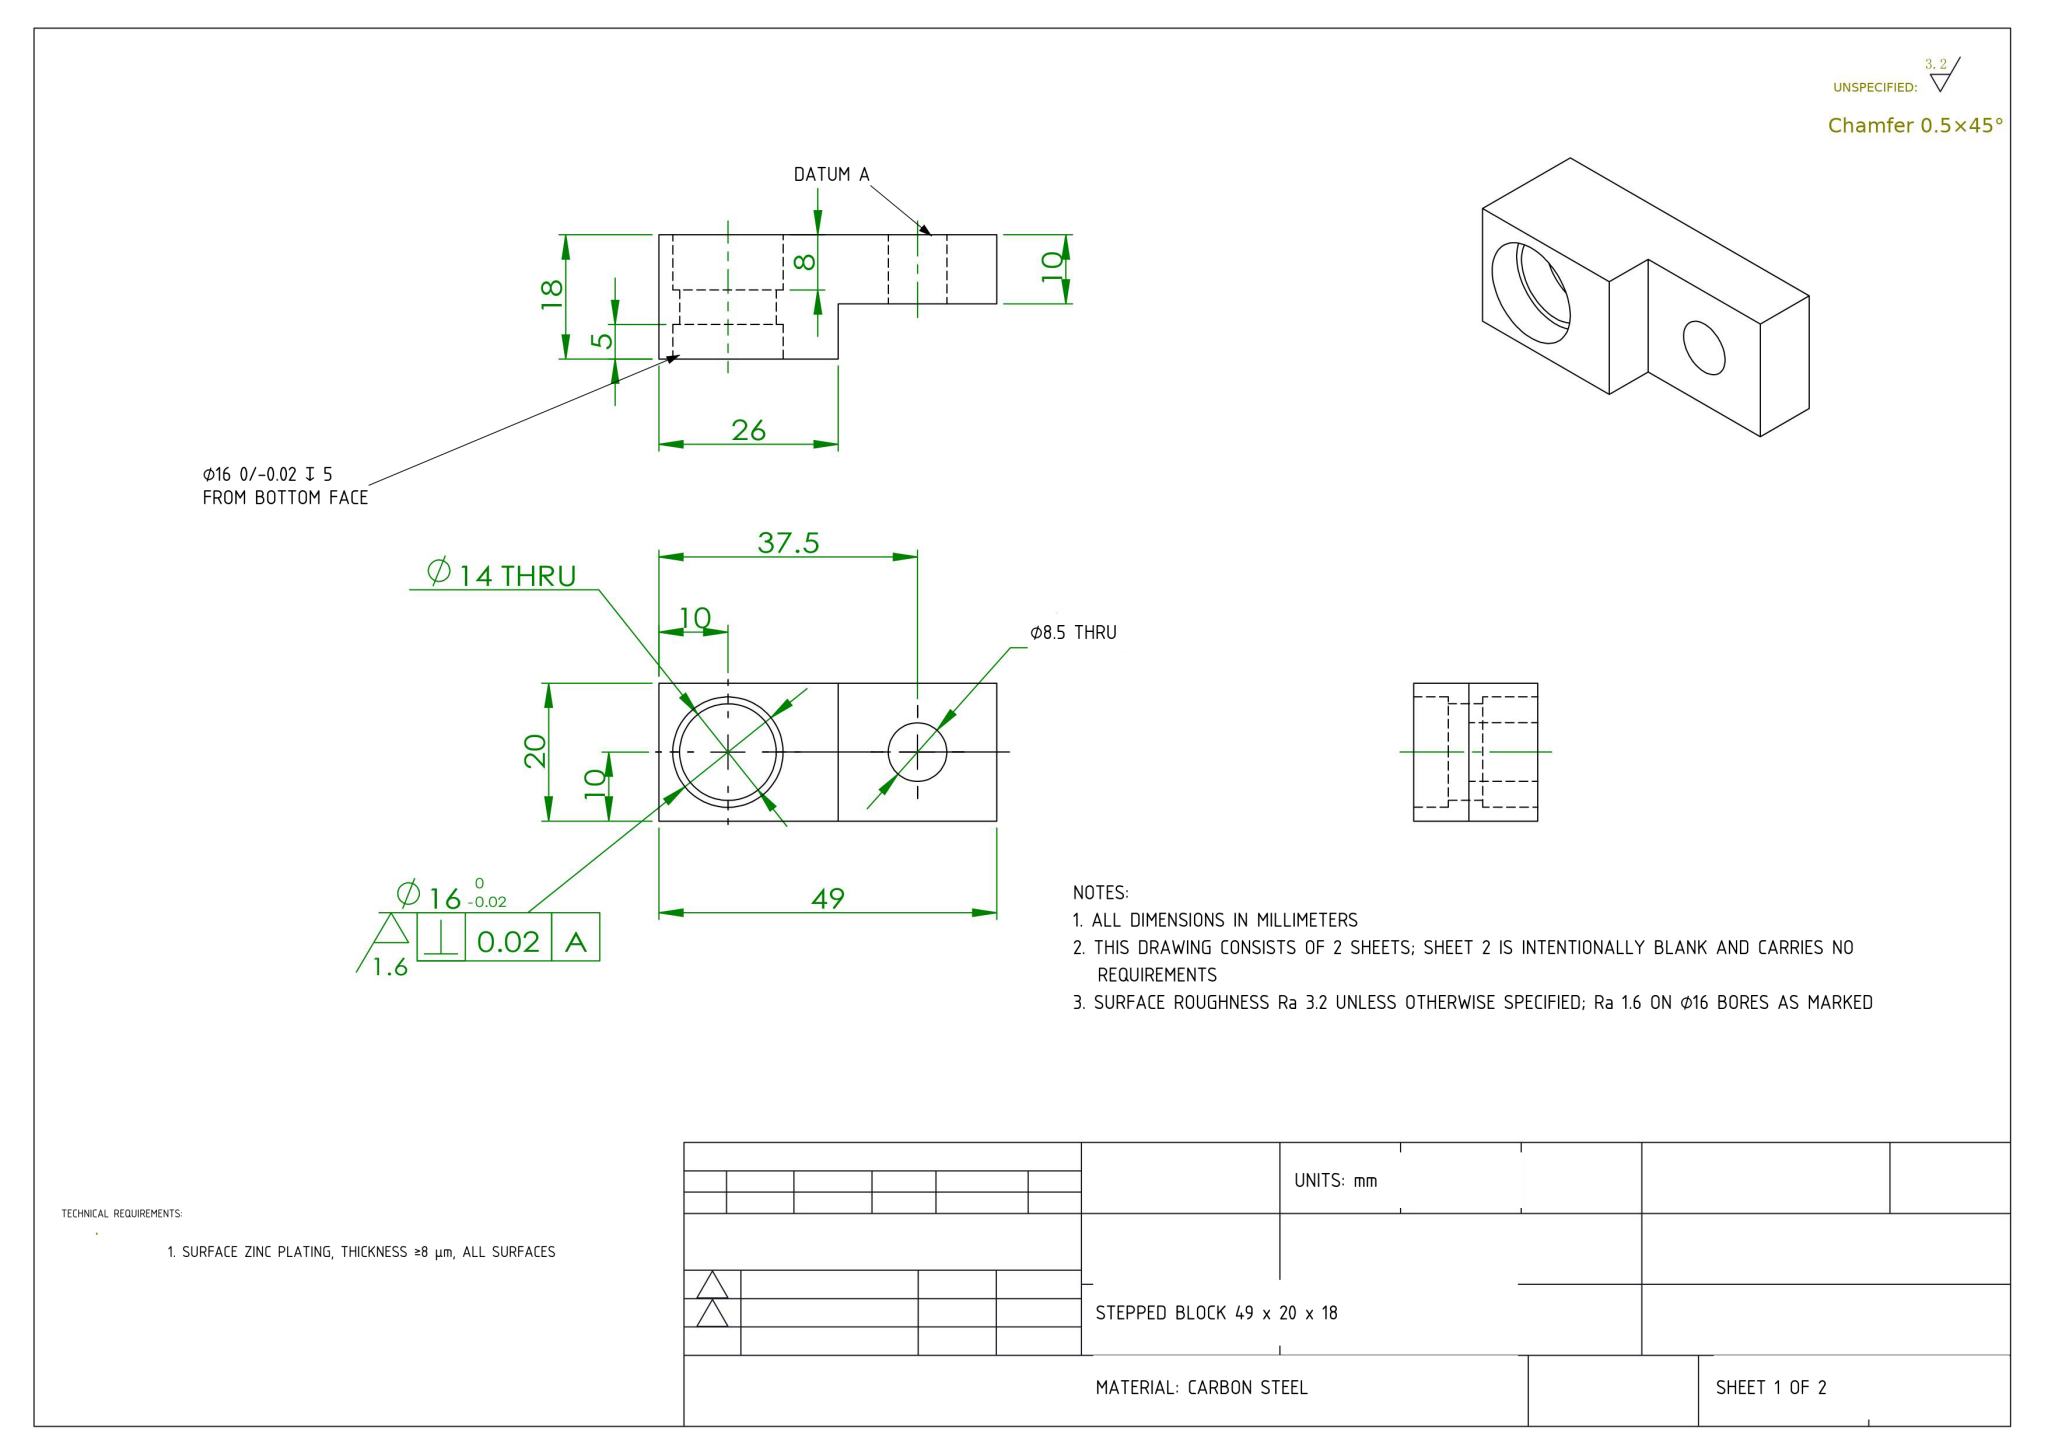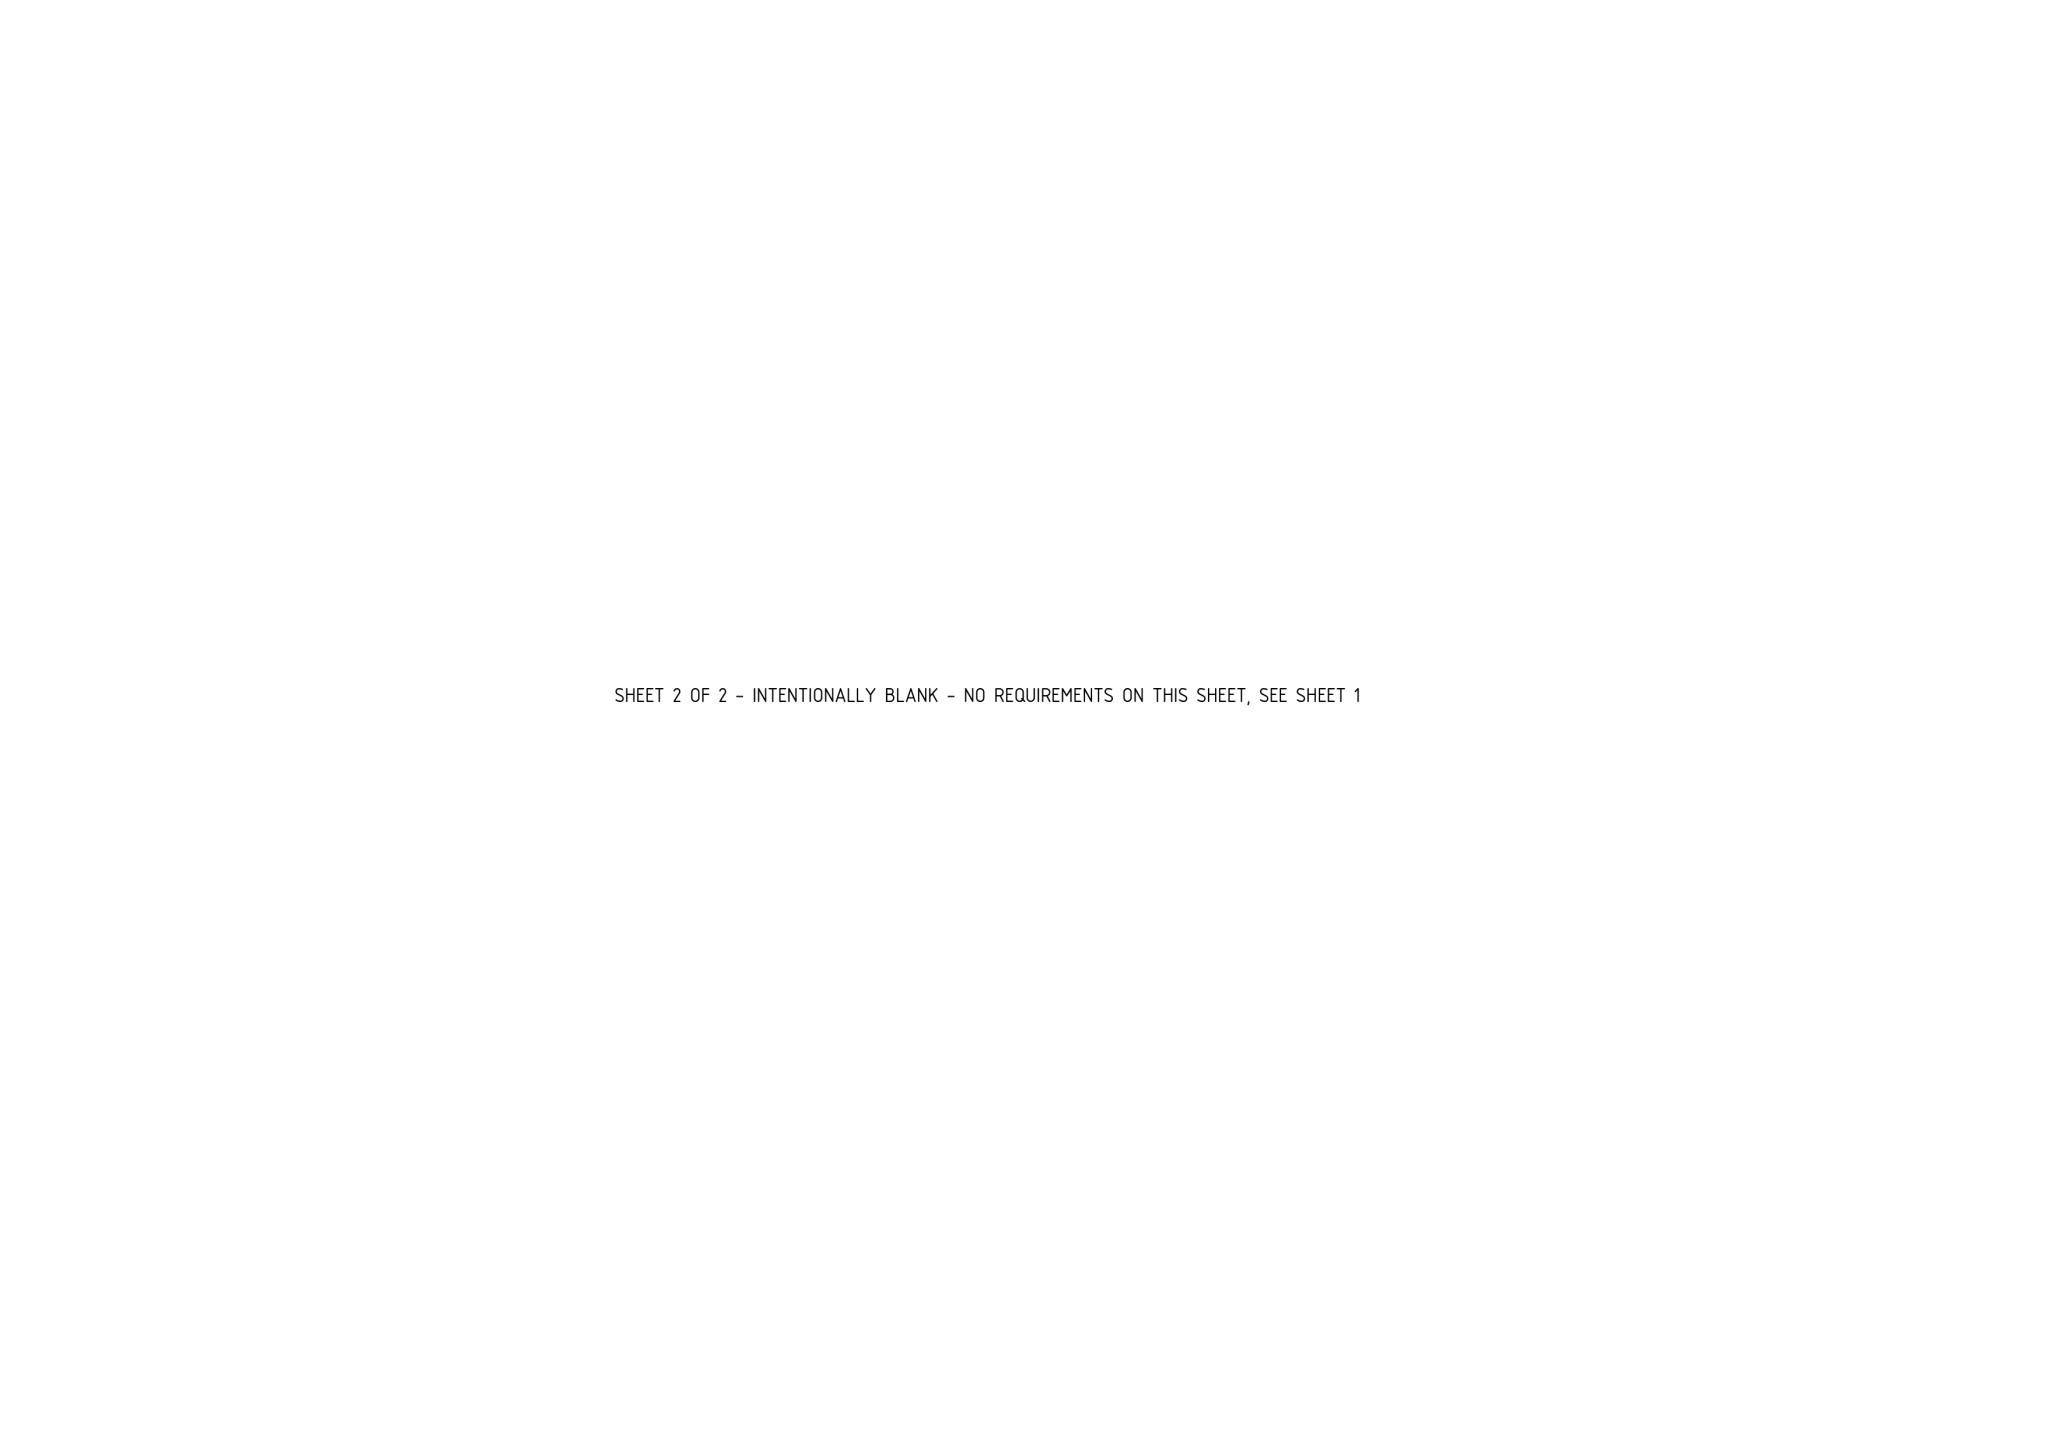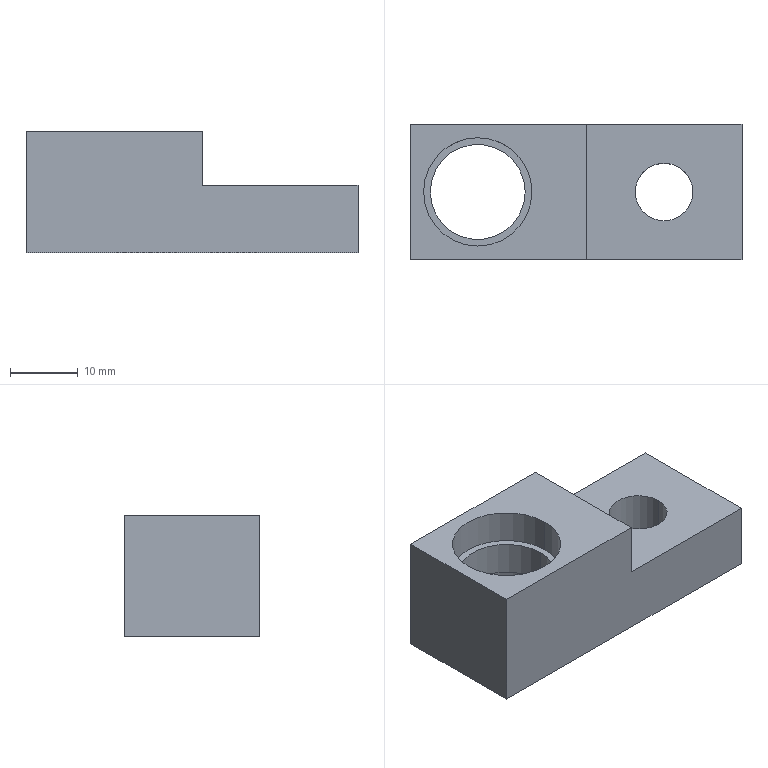Part | NX | mm | 1 solid | 18 faces | box 49 x 20 x 18 mm | volume 10009 mm3 | plane 10 | cylinder 8 | commonest cylinder face diameters 16 x4 8.5 x2 14 x2
STEP:
#1=COLOUR_RGB('',0.7961,0.8235,0.9373);
#2=FILL_AREA_STYLE_COLOUR('',#1);
#3=FILL_AREA_STYLE('',(#2));
#4=SURFACE_STYLE_FILL_AREA(#3);
#5=SURFACE_SIDE_STYLE('',(#4));
#6=SURFACE_STYLE_USAGE(.BOTH.,#5);
#7=PRESENTATION_STYLE_ASSIGNMENT((#6));
#8=CARTESIAN_POINT('',(18.,0.,8.));
#9=VERTEX_POINT('',#8);
#10=CARTESIAN_POINT('',(2.,0.,8.));
#11=VERTEX_POINT('',#10);
#12=CARTESIAN_POINT('',(10.,0.,8.));
#13=DIRECTION('',(0.,0.,-1.));
#14=DIRECTION('',(-1.,0.,0.));
#15=AXIS2_PLACEMENT_3D('',#12,#13,#14);
#16=CIRCLE('',#15,8.);
#17=EDGE_CURVE('',#9,#11,#16,.T.);
#18=ORIENTED_EDGE('',*,*,#17,.F.);
#19=CARTESIAN_POINT('',(18.,0.,0.));
#20=VERTEX_POINT('',#19);
#21=CARTESIAN_POINT('',(18.,0.,8.));
#22=DIRECTION('',(0.,0.,-1.));
#23=VECTOR('',#22,1000.);
#24=LINE('',#21,#23);
#25=EDGE_CURVE('',#9,#20,#24,.T.);
#26=ORIENTED_EDGE('',*,*,#25,.T.);
#27=CARTESIAN_POINT('',(2.,0.,0.));
#28=VERTEX_POINT('',#27);
#29=CARTESIAN_POINT('',(10.,0.,0.));
#30=DIRECTION('',(0.,0.,-1.));
#31=DIRECTION('',(-1.,0.,0.));
#32=AXIS2_PLACEMENT_3D('',#29,#30,#31);
#33=CIRCLE('',#32,8.);
#34=EDGE_CURVE('',#20,#28,#33,.T.);
#35=ORIENTED_EDGE('',*,*,#34,.T.);
#36=CARTESIAN_POINT('',(2.,0.,8.));
#37=DIRECTION('',(0.,0.,-1.));
#38=VECTOR('',#37,1000.);
#39=LINE('',#36,#38);
#40=EDGE_CURVE('',#11,#28,#39,.T.);
#41=ORIENTED_EDGE('',*,*,#40,.F.);
#42=EDGE_LOOP('',(#18,#26,#35,#41));
#43=FACE_OUTER_BOUND('',#42,.T.);
#44=CARTESIAN_POINT('',(10.,0.,8.));
#45=DIRECTION('',(0.,0.,-1.));
#46=DIRECTION('',(-1.,0.,0.));
#47=AXIS2_PLACEMENT_3D('',#44,#45,#46);
#48=CYLINDRICAL_SURFACE('',#47,8.);
#49=ADVANCED_FACE('',(#43),#48,.F.);
#50=CARTESIAN_POINT('',(2.,0.,13.));
#51=VERTEX_POINT('',#50);
#52=CARTESIAN_POINT('',(18.,0.,13.));
#53=VERTEX_POINT('',#52);
#54=CARTESIAN_POINT('',(10.,0.,13.));
#55=DIRECTION('',(0.,0.,1.));
#56=DIRECTION('',(1.,0.,0.));
#57=AXIS2_PLACEMENT_3D('',#54,#55,#56);
#58=CIRCLE('',#57,8.);
#59=EDGE_CURVE('',#51,#53,#58,.T.);
#60=ORIENTED_EDGE('',*,*,#59,.F.);
#61=CARTESIAN_POINT('',(2.,0.,18.));
#62=VERTEX_POINT('',#61);
#63=CARTESIAN_POINT('',(2.,0.,13.));
#64=DIRECTION('',(0.,0.,1.));
#65=VECTOR('',#64,1000.);
#66=LINE('',#63,#65);
#67=EDGE_CURVE('',#51,#62,#66,.T.);
#68=ORIENTED_EDGE('',*,*,#67,.T.);
#69=CARTESIAN_POINT('',(18.,0.,18.));
#70=VERTEX_POINT('',#69);
#71=CARTESIAN_POINT('',(10.,0.,18.));
#72=DIRECTION('',(0.,0.,1.));
#73=DIRECTION('',(1.,0.,0.));
#74=AXIS2_PLACEMENT_3D('',#71,#72,#73);
#75=CIRCLE('',#74,8.);
#76=EDGE_CURVE('',#62,#70,#75,.T.);
#77=ORIENTED_EDGE('',*,*,#76,.T.);
#78=CARTESIAN_POINT('',(18.,0.,13.));
#79=DIRECTION('',(0.,0.,1.));
#80=VECTOR('',#79,1000.);
#81=LINE('',#78,#80);
#82=EDGE_CURVE('',#53,#70,#81,.T.);
#83=ORIENTED_EDGE('',*,*,#82,.F.);
#84=EDGE_LOOP('',(#60,#68,#77,#83));
#85=FACE_OUTER_BOUND('',#84,.T.);
#86=CARTESIAN_POINT('',(10.,0.,13.));
#87=DIRECTION('',(0.,0.,1.));
#88=DIRECTION('',(1.,0.,0.));
#89=AXIS2_PLACEMENT_3D('',#86,#87,#88);
#90=CYLINDRICAL_SURFACE('',#89,8.);
#91=ADVANCED_FACE('',(#85),#90,.F.);
#92=CARTESIAN_POINT('',(33.25,0.,0.));
#93=VERTEX_POINT('',#92);
#94=CARTESIAN_POINT('',(41.75,0.,0.));
#95=VERTEX_POINT('',#94);
#96=CARTESIAN_POINT('',(37.5,0.,0.));
#97=DIRECTION('',(0.,0.,1.));
#98=DIRECTION('',(1.,0.,0.));
#99=AXIS2_PLACEMENT_3D('',#96,#97,#98);
#100=CIRCLE('',#99,4.25);
#101=EDGE_CURVE('',#93,#95,#100,.T.);
#102=ORIENTED_EDGE('',*,*,#101,.F.);
#103=CARTESIAN_POINT('',(33.25,0.,10.));
#104=VERTEX_POINT('',#103);
#105=CARTESIAN_POINT('',(33.25,0.,0.));
#106=DIRECTION('',(0.,0.,1.));
#107=VECTOR('',#106,1000.);
#108=LINE('',#105,#107);
#109=EDGE_CURVE('',#93,#104,#108,.T.);
#110=ORIENTED_EDGE('',*,*,#109,.T.);
#111=CARTESIAN_POINT('',(41.75,0.,10.));
#112=VERTEX_POINT('',#111);
#113=CARTESIAN_POINT('',(37.5,0.,10.));
#114=DIRECTION('',(0.,0.,1.));
#115=DIRECTION('',(1.,0.,0.));
#116=AXIS2_PLACEMENT_3D('',#113,#114,#115);
#117=CIRCLE('',#116,4.25);
#118=EDGE_CURVE('',#104,#112,#117,.T.);
#119=ORIENTED_EDGE('',*,*,#118,.T.);
#120=CARTESIAN_POINT('',(41.75,0.,0.));
#121=DIRECTION('',(0.,0.,1.));
#122=VECTOR('',#121,1000.);
#123=LINE('',#120,#122);
#124=EDGE_CURVE('',#95,#112,#123,.T.);
#125=ORIENTED_EDGE('',*,*,#124,.F.);
#126=EDGE_LOOP('',(#102,#110,#119,#125));
#127=FACE_OUTER_BOUND('',#126,.T.);
#128=CARTESIAN_POINT('',(37.5,0.,0.));
#129=DIRECTION('',(0.,0.,1.));
#130=DIRECTION('',(1.,0.,0.));
#131=AXIS2_PLACEMENT_3D('',#128,#129,#130);
#132=CYLINDRICAL_SURFACE('',#131,4.25);
#133=ADVANCED_FACE('',(#127),#132,.F.);
#134=CARTESIAN_POINT('',(3.,0.,8.));
#135=VERTEX_POINT('',#134);
#136=CARTESIAN_POINT('',(17.,0.,8.));
#137=VERTEX_POINT('',#136);
#138=CARTESIAN_POINT('',(10.,0.,8.));
#139=DIRECTION('',(0.,0.,1.));
#140=DIRECTION('',(-1.,0.,0.));
#141=AXIS2_PLACEMENT_3D('',#138,#139,#140);
#142=CIRCLE('',#141,7.);
#143=EDGE_CURVE('',#135,#137,#142,.T.);
#144=ORIENTED_EDGE('',*,*,#143,.F.);
#145=CARTESIAN_POINT('',(3.,0.,13.));
#146=VERTEX_POINT('',#145);
#147=CARTESIAN_POINT('',(3.,0.,0.));
#148=DIRECTION('',(0.,0.,1.));
#149=VECTOR('',#148,1000.);
#150=LINE('',#147,#149);
#151=EDGE_CURVE('',#135,#146,#150,.T.);
#152=ORIENTED_EDGE('',*,*,#151,.T.);
#153=CARTESIAN_POINT('',(17.,0.,13.));
#154=VERTEX_POINT('',#153);
#155=CARTESIAN_POINT('',(10.,0.,13.));
#156=DIRECTION('',(0.,0.,-1.));
#157=DIRECTION('',(1.,0.,0.));
#158=AXIS2_PLACEMENT_3D('',#155,#156,#157);
#159=CIRCLE('',#158,7.);
#160=EDGE_CURVE('',#154,#146,#159,.T.);
#161=ORIENTED_EDGE('',*,*,#160,.F.);
#162=CARTESIAN_POINT('',(17.,0.,0.));
#163=DIRECTION('',(0.,0.,1.));
#164=VECTOR('',#163,1000.);
#165=LINE('',#162,#164);
#166=EDGE_CURVE('',#137,#154,#165,.T.);
#167=ORIENTED_EDGE('',*,*,#166,.F.);
#168=EDGE_LOOP('',(#144,#152,#161,#167));
#169=FACE_OUTER_BOUND('',#168,.T.);
#170=CARTESIAN_POINT('',(10.,0.,0.));
#171=DIRECTION('',(0.,0.,1.));
#172=DIRECTION('',(1.,0.,0.));
#173=AXIS2_PLACEMENT_3D('',#170,#171,#172);
#174=CYLINDRICAL_SURFACE('',#173,7.);
#175=ADVANCED_FACE('',(#169),#174,.F.);
#176=ORIENTED_EDGE('',*,*,#151,.F.);
#177=CARTESIAN_POINT('',(10.,0.,8.));
#178=DIRECTION('',(0.,0.,1.));
#179=DIRECTION('',(-1.,0.,0.));
#180=AXIS2_PLACEMENT_3D('',#177,#178,#179);
#181=CIRCLE('',#180,7.);
#182=EDGE_CURVE('',#137,#135,#181,.T.);
#183=ORIENTED_EDGE('',*,*,#182,.F.);
#184=ORIENTED_EDGE('',*,*,#166,.T.);
#185=CARTESIAN_POINT('',(10.,0.,13.));
#186=DIRECTION('',(0.,0.,-1.));
#187=DIRECTION('',(1.,0.,0.));
#188=AXIS2_PLACEMENT_3D('',#185,#186,#187);
#189=CIRCLE('',#188,7.);
#190=EDGE_CURVE('',#146,#154,#189,.T.);
#191=ORIENTED_EDGE('',*,*,#190,.F.);
#192=EDGE_LOOP('',(#176,#183,#184,#191));
#193=FACE_OUTER_BOUND('',#192,.T.);
#194=CARTESIAN_POINT('',(10.,0.,0.));
#195=DIRECTION('',(0.,0.,1.));
#196=DIRECTION('',(1.,0.,0.));
#197=AXIS2_PLACEMENT_3D('',#194,#195,#196);
#198=CYLINDRICAL_SURFACE('',#197,7.);
#199=ADVANCED_FACE('',(#193),#198,.F.);
#200=CARTESIAN_POINT('',(0.,-10.,0.));
#201=VERTEX_POINT('',#200);
#202=CARTESIAN_POINT('',(0.,-10.,18.));
#203=VERTEX_POINT('',#202);
#204=CARTESIAN_POINT('',(0.,-10.,18.));
#205=DIRECTION('',(0.,0.,1.));
#206=VECTOR('',#205,1000.);
#207=LINE('',#204,#206);
#208=EDGE_CURVE('',#201,#203,#207,.T.);
#209=ORIENTED_EDGE('',*,*,#208,.T.);
#210=CARTESIAN_POINT('',(0.,10.,18.));
#211=VERTEX_POINT('',#210);
#212=CARTESIAN_POINT('',(0.,10.,18.));
#213=DIRECTION('',(0.,-1.,0.));
#214=VECTOR('',#213,1000.);
#215=LINE('',#212,#214);
#216=EDGE_CURVE('',#211,#203,#215,.T.);
#217=ORIENTED_EDGE('',*,*,#216,.F.);
#218=CARTESIAN_POINT('',(0.,10.,0.));
#219=VERTEX_POINT('',#218);
#220=CARTESIAN_POINT('',(0.,10.,18.));
#221=DIRECTION('',(0.,0.,1.));
#222=VECTOR('',#221,1000.);
#223=LINE('',#220,#222);
#224=EDGE_CURVE('',#219,#211,#223,.T.);
#225=ORIENTED_EDGE('',*,*,#224,.F.);
#226=CARTESIAN_POINT('',(0.,10.,0.));
#227=DIRECTION('',(0.,-1.,0.));
#228=VECTOR('',#227,1000.);
#229=LINE('',#226,#228);
#230=EDGE_CURVE('',#219,#201,#229,.T.);
#231=ORIENTED_EDGE('',*,*,#230,.T.);
#232=EDGE_LOOP('',(#209,#217,#225,#231));
#233=FACE_OUTER_BOUND('',#232,.T.);
#234=CARTESIAN_POINT('',(0.,10.,18.));
#235=DIRECTION('',(1.,0.,-0.));
#236=DIRECTION('',(-0.,0.,-1.));
#237=AXIS2_PLACEMENT_3D('',#234,#235,#236);
#238=PLANE('',#237);
#239=ADVANCED_FACE('',(#233),#238,.F.);
#240=CARTESIAN_POINT('',(10.,0.,18.));
#241=DIRECTION('',(0.,0.,1.));
#242=DIRECTION('',(1.,0.,0.));
#243=AXIS2_PLACEMENT_3D('',#240,#241,#242);
#244=CIRCLE('',#243,8.);
#245=EDGE_CURVE('',#70,#62,#244,.T.);
#246=ORIENTED_EDGE('',*,*,#245,.F.);
#247=ORIENTED_EDGE('',*,*,#76,.F.);
#248=EDGE_LOOP('',(#246,#247));
#249=FACE_BOUND('',#248,.T.);
#250=CARTESIAN_POINT('',(26.,-10.,18.));
#251=VERTEX_POINT('',#250);
#252=CARTESIAN_POINT('',(26.,-10.,18.));
#253=DIRECTION('',(1.,0.,-0.));
#254=VECTOR('',#253,1000.);
#255=LINE('',#252,#254);
#256=EDGE_CURVE('',#203,#251,#255,.T.);
#257=ORIENTED_EDGE('',*,*,#256,.T.);
#258=CARTESIAN_POINT('',(26.,10.,18.));
#259=VERTEX_POINT('',#258);
#260=CARTESIAN_POINT('',(26.,10.,18.));
#261=DIRECTION('',(0.,-1.,0.));
#262=VECTOR('',#261,1000.);
#263=LINE('',#260,#262);
#264=EDGE_CURVE('',#259,#251,#263,.T.);
#265=ORIENTED_EDGE('',*,*,#264,.F.);
#266=CARTESIAN_POINT('',(26.,10.,18.));
#267=DIRECTION('',(1.,0.,-0.));
#268=VECTOR('',#267,1000.);
#269=LINE('',#266,#268);
#270=EDGE_CURVE('',#211,#259,#269,.T.);
#271=ORIENTED_EDGE('',*,*,#270,.F.);
#272=ORIENTED_EDGE('',*,*,#216,.T.);
#273=EDGE_LOOP('',(#257,#265,#271,#272));
#274=FACE_OUTER_BOUND('',#273,.T.);
#275=CARTESIAN_POINT('',(26.,10.,18.));
#276=DIRECTION('',(-0.,0.,-1.));
#277=DIRECTION('',(-1.,0.,0.));
#278=AXIS2_PLACEMENT_3D('',#275,#276,#277);
#279=PLANE('',#278);
#280=ADVANCED_FACE('',(#249,#274),#279,.F.);
#281=CARTESIAN_POINT('',(26.,-10.,10.));
#282=VERTEX_POINT('',#281);
#283=CARTESIAN_POINT('',(26.,-10.,10.));
#284=DIRECTION('',(-0.,0.,-1.));
#285=VECTOR('',#284,1000.);
#286=LINE('',#283,#285);
#287=EDGE_CURVE('',#251,#282,#286,.T.);
#288=ORIENTED_EDGE('',*,*,#287,.T.);
#289=CARTESIAN_POINT('',(26.,10.,10.));
#290=VERTEX_POINT('',#289);
#291=CARTESIAN_POINT('',(26.,10.,10.));
#292=DIRECTION('',(0.,-1.,0.));
#293=VECTOR('',#292,1000.);
#294=LINE('',#291,#293);
#295=EDGE_CURVE('',#290,#282,#294,.T.);
#296=ORIENTED_EDGE('',*,*,#295,.F.);
#297=CARTESIAN_POINT('',(26.,10.,10.));
#298=DIRECTION('',(-0.,0.,-1.));
#299=VECTOR('',#298,1000.);
#300=LINE('',#297,#299);
#301=EDGE_CURVE('',#259,#290,#300,.T.);
#302=ORIENTED_EDGE('',*,*,#301,.F.);
#303=ORIENTED_EDGE('',*,*,#264,.T.);
#304=EDGE_LOOP('',(#288,#296,#302,#303));
#305=FACE_OUTER_BOUND('',#304,.T.);
#306=CARTESIAN_POINT('',(26.,10.,10.));
#307=DIRECTION('',(-1.,0.,0.));
#308=DIRECTION('',(0.,0.,1.));
#309=AXIS2_PLACEMENT_3D('',#306,#307,#308);
#310=PLANE('',#309);
#311=ADVANCED_FACE('',(#305),#310,.F.);
#312=CARTESIAN_POINT('',(37.5,0.,10.));
#313=DIRECTION('',(0.,0.,1.));
#314=DIRECTION('',(1.,0.,0.));
#315=AXIS2_PLACEMENT_3D('',#312,#313,#314);
#316=CIRCLE('',#315,4.25);
#317=EDGE_CURVE('',#112,#104,#316,.T.);
#318=ORIENTED_EDGE('',*,*,#317,.F.);
#319=ORIENTED_EDGE('',*,*,#118,.F.);
#320=EDGE_LOOP('',(#318,#319));
#321=FACE_BOUND('',#320,.T.);
#322=CARTESIAN_POINT('',(49.,-10.,10.));
#323=VERTEX_POINT('',#322);
#324=CARTESIAN_POINT('',(49.,-10.,10.));
#325=DIRECTION('',(1.,0.,-0.));
#326=VECTOR('',#325,1000.);
#327=LINE('',#324,#326);
#328=EDGE_CURVE('',#282,#323,#327,.T.);
#329=ORIENTED_EDGE('',*,*,#328,.T.);
#330=CARTESIAN_POINT('',(49.,10.,10.));
#331=VERTEX_POINT('',#330);
#332=CARTESIAN_POINT('',(49.,10.,10.));
#333=DIRECTION('',(0.,-1.,0.));
#334=VECTOR('',#333,1000.);
#335=LINE('',#332,#334);
#336=EDGE_CURVE('',#331,#323,#335,.T.);
#337=ORIENTED_EDGE('',*,*,#336,.F.);
#338=CARTESIAN_POINT('',(49.,10.,10.));
#339=DIRECTION('',(1.,0.,-0.));
#340=VECTOR('',#339,1000.);
#341=LINE('',#338,#340);
#342=EDGE_CURVE('',#290,#331,#341,.T.);
#343=ORIENTED_EDGE('',*,*,#342,.F.);
#344=ORIENTED_EDGE('',*,*,#295,.T.);
#345=EDGE_LOOP('',(#329,#337,#343,#344));
#346=FACE_OUTER_BOUND('',#345,.T.);
#347=CARTESIAN_POINT('',(49.,10.,10.));
#348=DIRECTION('',(-0.,0.,-1.));
#349=DIRECTION('',(-1.,0.,0.));
#350=AXIS2_PLACEMENT_3D('',#347,#348,#349);
#351=PLANE('',#350);
#352=ADVANCED_FACE('',(#321,#346),#351,.F.);
#353=CARTESIAN_POINT('',(49.,-10.,0.));
#354=VERTEX_POINT('',#353);
#355=CARTESIAN_POINT('',(49.,-10.,0.));
#356=DIRECTION('',(0.,0.,-1.));
#357=VECTOR('',#356,1000.);
#358=LINE('',#355,#357);
#359=EDGE_CURVE('',#323,#354,#358,.T.);
#360=ORIENTED_EDGE('',*,*,#359,.T.);
#361=CARTESIAN_POINT('',(49.,10.,0.));
#362=VERTEX_POINT('',#361);
#363=CARTESIAN_POINT('',(49.,10.,0.));
#364=DIRECTION('',(0.,-1.,0.));
#365=VECTOR('',#364,1000.);
#366=LINE('',#363,#365);
#367=EDGE_CURVE('',#362,#354,#366,.T.);
#368=ORIENTED_EDGE('',*,*,#367,.F.);
#369=CARTESIAN_POINT('',(49.,10.,0.));
#370=DIRECTION('',(0.,0.,-1.));
#371=VECTOR('',#370,1000.);
#372=LINE('',#369,#371);
#373=EDGE_CURVE('',#331,#362,#372,.T.);
#374=ORIENTED_EDGE('',*,*,#373,.F.);
#375=ORIENTED_EDGE('',*,*,#336,.T.);
#376=EDGE_LOOP('',(#360,#368,#374,#375));
#377=FACE_OUTER_BOUND('',#376,.T.);
#378=CARTESIAN_POINT('',(49.,10.,0.));
#379=DIRECTION('',(-1.,0.,0.));
#380=DIRECTION('',(0.,0.,1.));
#381=AXIS2_PLACEMENT_3D('',#378,#379,#380);
#382=PLANE('',#381);
#383=ADVANCED_FACE('',(#377),#382,.F.);
#384=CARTESIAN_POINT('',(10.,0.,0.));
#385=DIRECTION('',(0.,0.,-1.));
#386=DIRECTION('',(-1.,0.,0.));
#387=AXIS2_PLACEMENT_3D('',#384,#385,#386);
#388=CIRCLE('',#387,8.);
#389=EDGE_CURVE('',#28,#20,#388,.T.);
#390=ORIENTED_EDGE('',*,*,#389,.F.);
#391=ORIENTED_EDGE('',*,*,#34,.F.);
#392=EDGE_LOOP('',(#390,#391));
#393=FACE_BOUND('',#392,.T.);
#394=CARTESIAN_POINT('',(37.5,0.,0.));
#395=DIRECTION('',(0.,0.,1.));
#396=DIRECTION('',(1.,0.,0.));
#397=AXIS2_PLACEMENT_3D('',#394,#395,#396);
#398=CIRCLE('',#397,4.25);
#399=EDGE_CURVE('',#95,#93,#398,.T.);
#400=ORIENTED_EDGE('',*,*,#399,.T.);
#401=ORIENTED_EDGE('',*,*,#101,.T.);
#402=EDGE_LOOP('',(#400,#401));
#403=FACE_BOUND('',#402,.T.);
#404=CARTESIAN_POINT('',(0.,-10.,0.));
#405=DIRECTION('',(-1.,0.,0.));
#406=VECTOR('',#405,1000.);
#407=LINE('',#404,#406);
#408=EDGE_CURVE('',#354,#201,#407,.T.);
#409=ORIENTED_EDGE('',*,*,#408,.T.);
#410=ORIENTED_EDGE('',*,*,#230,.F.);
#411=CARTESIAN_POINT('',(0.,10.,0.));
#412=DIRECTION('',(-1.,0.,0.));
#413=VECTOR('',#412,1000.);
#414=LINE('',#411,#413);
#415=EDGE_CURVE('',#362,#219,#414,.T.);
#416=ORIENTED_EDGE('',*,*,#415,.F.);
#417=ORIENTED_EDGE('',*,*,#367,.T.);
#418=EDGE_LOOP('',(#409,#410,#416,#417));
#419=FACE_OUTER_BOUND('',#418,.T.);
#420=CARTESIAN_POINT('',(0.,10.,0.));
#421=DIRECTION('',(0.,0.,1.));
#422=DIRECTION('',(1.,0.,0.));
#423=AXIS2_PLACEMENT_3D('',#420,#421,#422);
#424=PLANE('',#423);
#425=ADVANCED_FACE('',(#393,#403,#419),#424,.F.);
#426=ORIENTED_EDGE('',*,*,#224,.T.);
#427=ORIENTED_EDGE('',*,*,#270,.T.);
#428=ORIENTED_EDGE('',*,*,#301,.T.);
#429=ORIENTED_EDGE('',*,*,#342,.T.);
#430=ORIENTED_EDGE('',*,*,#373,.T.);
#431=ORIENTED_EDGE('',*,*,#415,.T.);
#432=EDGE_LOOP('',(#426,#427,#428,#429,#430,#431));
#433=FACE_OUTER_BOUND('',#432,.T.);
#434=CARTESIAN_POINT('',(0.,10.,10.));
#435=DIRECTION('',(0.,1.,0.));
#436=DIRECTION('',(0.,0.,1.));
#437=AXIS2_PLACEMENT_3D('',#434,#435,#436);
#438=PLANE('',#437);
#439=ADVANCED_FACE('',(#433),#438,.T.);
#440=ORIENTED_EDGE('',*,*,#208,.F.);
#441=ORIENTED_EDGE('',*,*,#408,.F.);
#442=ORIENTED_EDGE('',*,*,#359,.F.);
#443=ORIENTED_EDGE('',*,*,#328,.F.);
#444=ORIENTED_EDGE('',*,*,#287,.F.);
#445=ORIENTED_EDGE('',*,*,#256,.F.);
#446=EDGE_LOOP('',(#440,#441,#442,#443,#444,#445));
#447=FACE_OUTER_BOUND('',#446,.T.);
#448=CARTESIAN_POINT('',(0.,-10.,10.));
#449=DIRECTION('',(0.,1.,0.));
#450=DIRECTION('',(0.,0.,1.));
#451=AXIS2_PLACEMENT_3D('',#448,#449,#450);
#452=PLANE('',#451);
#453=ADVANCED_FACE('',(#447),#452,.F.);
#454=ORIENTED_EDGE('',*,*,#109,.F.);
#455=ORIENTED_EDGE('',*,*,#399,.F.);
#456=ORIENTED_EDGE('',*,*,#124,.T.);
#457=ORIENTED_EDGE('',*,*,#317,.T.);
#458=EDGE_LOOP('',(#454,#455,#456,#457));
#459=FACE_OUTER_BOUND('',#458,.T.);
#460=CARTESIAN_POINT('',(37.5,0.,0.));
#461=DIRECTION('',(0.,0.,1.));
#462=DIRECTION('',(1.,0.,0.));
#463=AXIS2_PLACEMENT_3D('',#460,#461,#462);
#464=CYLINDRICAL_SURFACE('',#463,4.25);
#465=ADVANCED_FACE('',(#459),#464,.F.);
#466=CARTESIAN_POINT('',(10.,0.,13.));
#467=DIRECTION('',(0.,0.,1.));
#468=DIRECTION('',(1.,0.,0.));
#469=AXIS2_PLACEMENT_3D('',#466,#467,#468);
#470=CIRCLE('',#469,8.);
#471=EDGE_CURVE('',#53,#51,#470,.T.);
#472=ORIENTED_EDGE('',*,*,#471,.T.);
#473=ORIENTED_EDGE('',*,*,#59,.T.);
#474=EDGE_LOOP('',(#472,#473));
#475=FACE_OUTER_BOUND('',#474,.T.);
#476=ORIENTED_EDGE('',*,*,#160,.T.);
#477=ORIENTED_EDGE('',*,*,#190,.T.);
#478=EDGE_LOOP('',(#476,#477));
#479=FACE_BOUND('',#478,.T.);
#480=CARTESIAN_POINT('',(10.,0.,13.));
#481=DIRECTION('',(0.,0.,1.));
#482=DIRECTION('',(1.,0.,0.));
#483=AXIS2_PLACEMENT_3D('',#480,#481,#482);
#484=PLANE('',#483);
#485=ADVANCED_FACE('',(#475,#479),#484,.T.);
#486=ORIENTED_EDGE('',*,*,#67,.F.);
#487=ORIENTED_EDGE('',*,*,#471,.F.);
#488=ORIENTED_EDGE('',*,*,#82,.T.);
#489=ORIENTED_EDGE('',*,*,#245,.T.);
#490=EDGE_LOOP('',(#486,#487,#488,#489));
#491=FACE_OUTER_BOUND('',#490,.T.);
#492=CARTESIAN_POINT('',(10.,0.,13.));
#493=DIRECTION('',(0.,0.,1.));
#494=DIRECTION('',(1.,0.,0.));
#495=AXIS2_PLACEMENT_3D('',#492,#493,#494);
#496=CYLINDRICAL_SURFACE('',#495,8.);
#497=ADVANCED_FACE('',(#491),#496,.F.);
#498=CARTESIAN_POINT('',(10.,0.,8.));
#499=DIRECTION('',(0.,0.,-1.));
#500=DIRECTION('',(-1.,0.,0.));
#501=AXIS2_PLACEMENT_3D('',#498,#499,#500);
#502=CIRCLE('',#501,8.);
#503=EDGE_CURVE('',#11,#9,#502,.T.);
#504=ORIENTED_EDGE('',*,*,#503,.T.);
#505=ORIENTED_EDGE('',*,*,#17,.T.);
#506=EDGE_LOOP('',(#504,#505));
#507=FACE_OUTER_BOUND('',#506,.T.);
#508=ORIENTED_EDGE('',*,*,#182,.T.);
#509=ORIENTED_EDGE('',*,*,#143,.T.);
#510=EDGE_LOOP('',(#508,#509));
#511=FACE_BOUND('',#510,.T.);
#512=CARTESIAN_POINT('',(10.,0.,8.));
#513=DIRECTION('',(0.,0.,-1.));
#514=DIRECTION('',(-1.,0.,0.));
#515=AXIS2_PLACEMENT_3D('',#512,#513,#514);
#516=PLANE('',#515);
#517=ADVANCED_FACE('',(#507,#511),#516,.T.);
#518=ORIENTED_EDGE('',*,*,#25,.F.);
#519=ORIENTED_EDGE('',*,*,#503,.F.);
#520=ORIENTED_EDGE('',*,*,#40,.T.);
#521=ORIENTED_EDGE('',*,*,#389,.T.);
#522=EDGE_LOOP('',(#518,#519,#520,#521));
#523=FACE_OUTER_BOUND('',#522,.T.);
#524=CARTESIAN_POINT('',(10.,0.,8.));
#525=DIRECTION('',(0.,0.,-1.));
#526=DIRECTION('',(-1.,0.,0.));
#527=AXIS2_PLACEMENT_3D('',#524,#525,#526);
#528=CYLINDRICAL_SURFACE('',#527,8.);
#529=ADVANCED_FACE('',(#523),#528,.F.);
#530=CLOSED_SHELL('',(#49,#91,#133,#175,#199,#239,#280,#311,#352,#383,#425,#439,#453,#465,#485,#497,#517,#529));
#531=MANIFOLD_SOLID_BREP('',#530);
#532=STYLED_ITEM('',(#7),#531);
#533=(LENGTH_UNIT()NAMED_UNIT(*)SI_UNIT(.MILLI.,.METRE.));
#534=UNCERTAINTY_MEASURE_WITH_UNIT(LENGTH_MEASURE(0.00001),#533,'','');
#535=(NAMED_UNIT(*)PLANE_ANGLE_UNIT()SI_UNIT($,.RADIAN.));
#536=(NAMED_UNIT(*)SI_UNIT($,.STERADIAN.)SOLID_ANGLE_UNIT());
#537=(GEOMETRIC_REPRESENTATION_CONTEXT(3)GLOBAL_UNCERTAINTY_ASSIGNED_CONTEXT((#534))GLOBAL_UNIT_ASSIGNED_CONTEXT((#533,#535,#536))REPRESENTATION_CONTEXT('',''));
#538=MECHANICAL_DESIGN_GEOMETRIC_PRESENTATION_REPRESENTATION('',(#532),#537);
#539=PRESENTATION_LAYER_ASSIGNMENT('','',(#532));
#540=COLOUR_RGB('',0.7961,0.8235,0.9373);
#541=FILL_AREA_STYLE_COLOUR('',#540);
#542=FILL_AREA_STYLE('',(#541));
#543=SURFACE_STYLE_FILL_AREA(#542);
#544=SURFACE_SIDE_STYLE('',(#543));
#545=SURFACE_STYLE_USAGE(.BOTH.,#544);
#546=PRESENTATION_STYLE_ASSIGNMENT((#545));
#547=CARTESIAN_POINT('',(0.,0.,0.));
#548=DIRECTION('',(0.,0.,1.));
#549=DIRECTION('',(1.,0.,0.));
#550=AXIS2_PLACEMENT_3D('',#547,#548,#549);
#551=(LENGTH_UNIT()NAMED_UNIT(*)SI_UNIT(.MILLI.,.METRE.));
#552=UNCERTAINTY_MEASURE_WITH_UNIT(LENGTH_MEASURE(0.00001),#551,'','');
#553=(NAMED_UNIT(*)PLANE_ANGLE_UNIT()SI_UNIT($,.RADIAN.));
#554=(NAMED_UNIT(*)SI_UNIT($,.STERADIAN.)SOLID_ANGLE_UNIT());
#555=(GEOMETRIC_REPRESENTATION_CONTEXT(3)GLOBAL_UNCERTAINTY_ASSIGNED_CONTEXT((#552))GLOBAL_UNIT_ASSIGNED_CONTEXT((#551,#553,#554))REPRESENTATION_CONTEXT('',''));
#556=ADVANCED_BREP_SHAPE_REPRESENTATION('',(#531,#550),#555);
#557=STYLED_ITEM('',(#546),#556);
#558=PRESENTATION_LAYER_ASSIGNMENT('','',(#557));
#559=(LENGTH_UNIT()NAMED_UNIT(*)SI_UNIT(.MILLI.,.METRE.));
#560=UNCERTAINTY_MEASURE_WITH_UNIT(LENGTH_MEASURE(0.00001),#559,'','');
#561=(NAMED_UNIT(*)PLANE_ANGLE_UNIT()SI_UNIT($,.RADIAN.));
#562=(NAMED_UNIT(*)SI_UNIT($,.STERADIAN.)SOLID_ANGLE_UNIT());
#563=(GEOMETRIC_REPRESENTATION_CONTEXT(3)GLOBAL_UNCERTAINTY_ASSIGNED_CONTEXT((#560))GLOBAL_UNIT_ASSIGNED_CONTEXT((#559,#561,#562))REPRESENTATION_CONTEXT('',''));
#564=MECHANICAL_DESIGN_GEOMETRIC_PRESENTATION_REPRESENTATION('',(#557),#563);